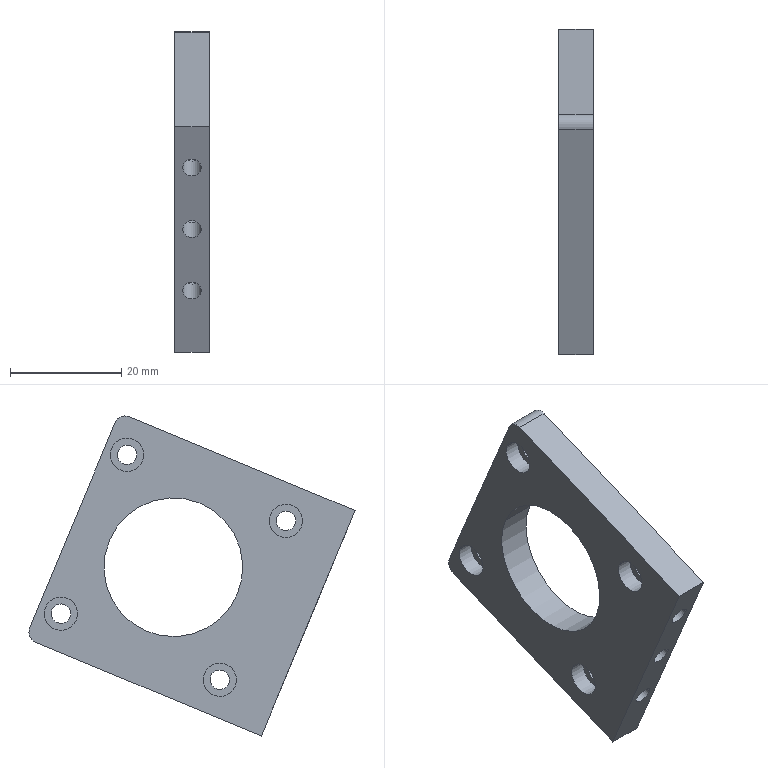Component | SolidWorks | CuttingInductionSeat16-1-2 | 1 solid | 42 faces | volume 8844 mm3 | cylinder 26 | plane 10 | cone 6 | commonest cylinder face diameters 6 x8 3.5 x8 3.3 x6 25 x2 4 x2 | material A3